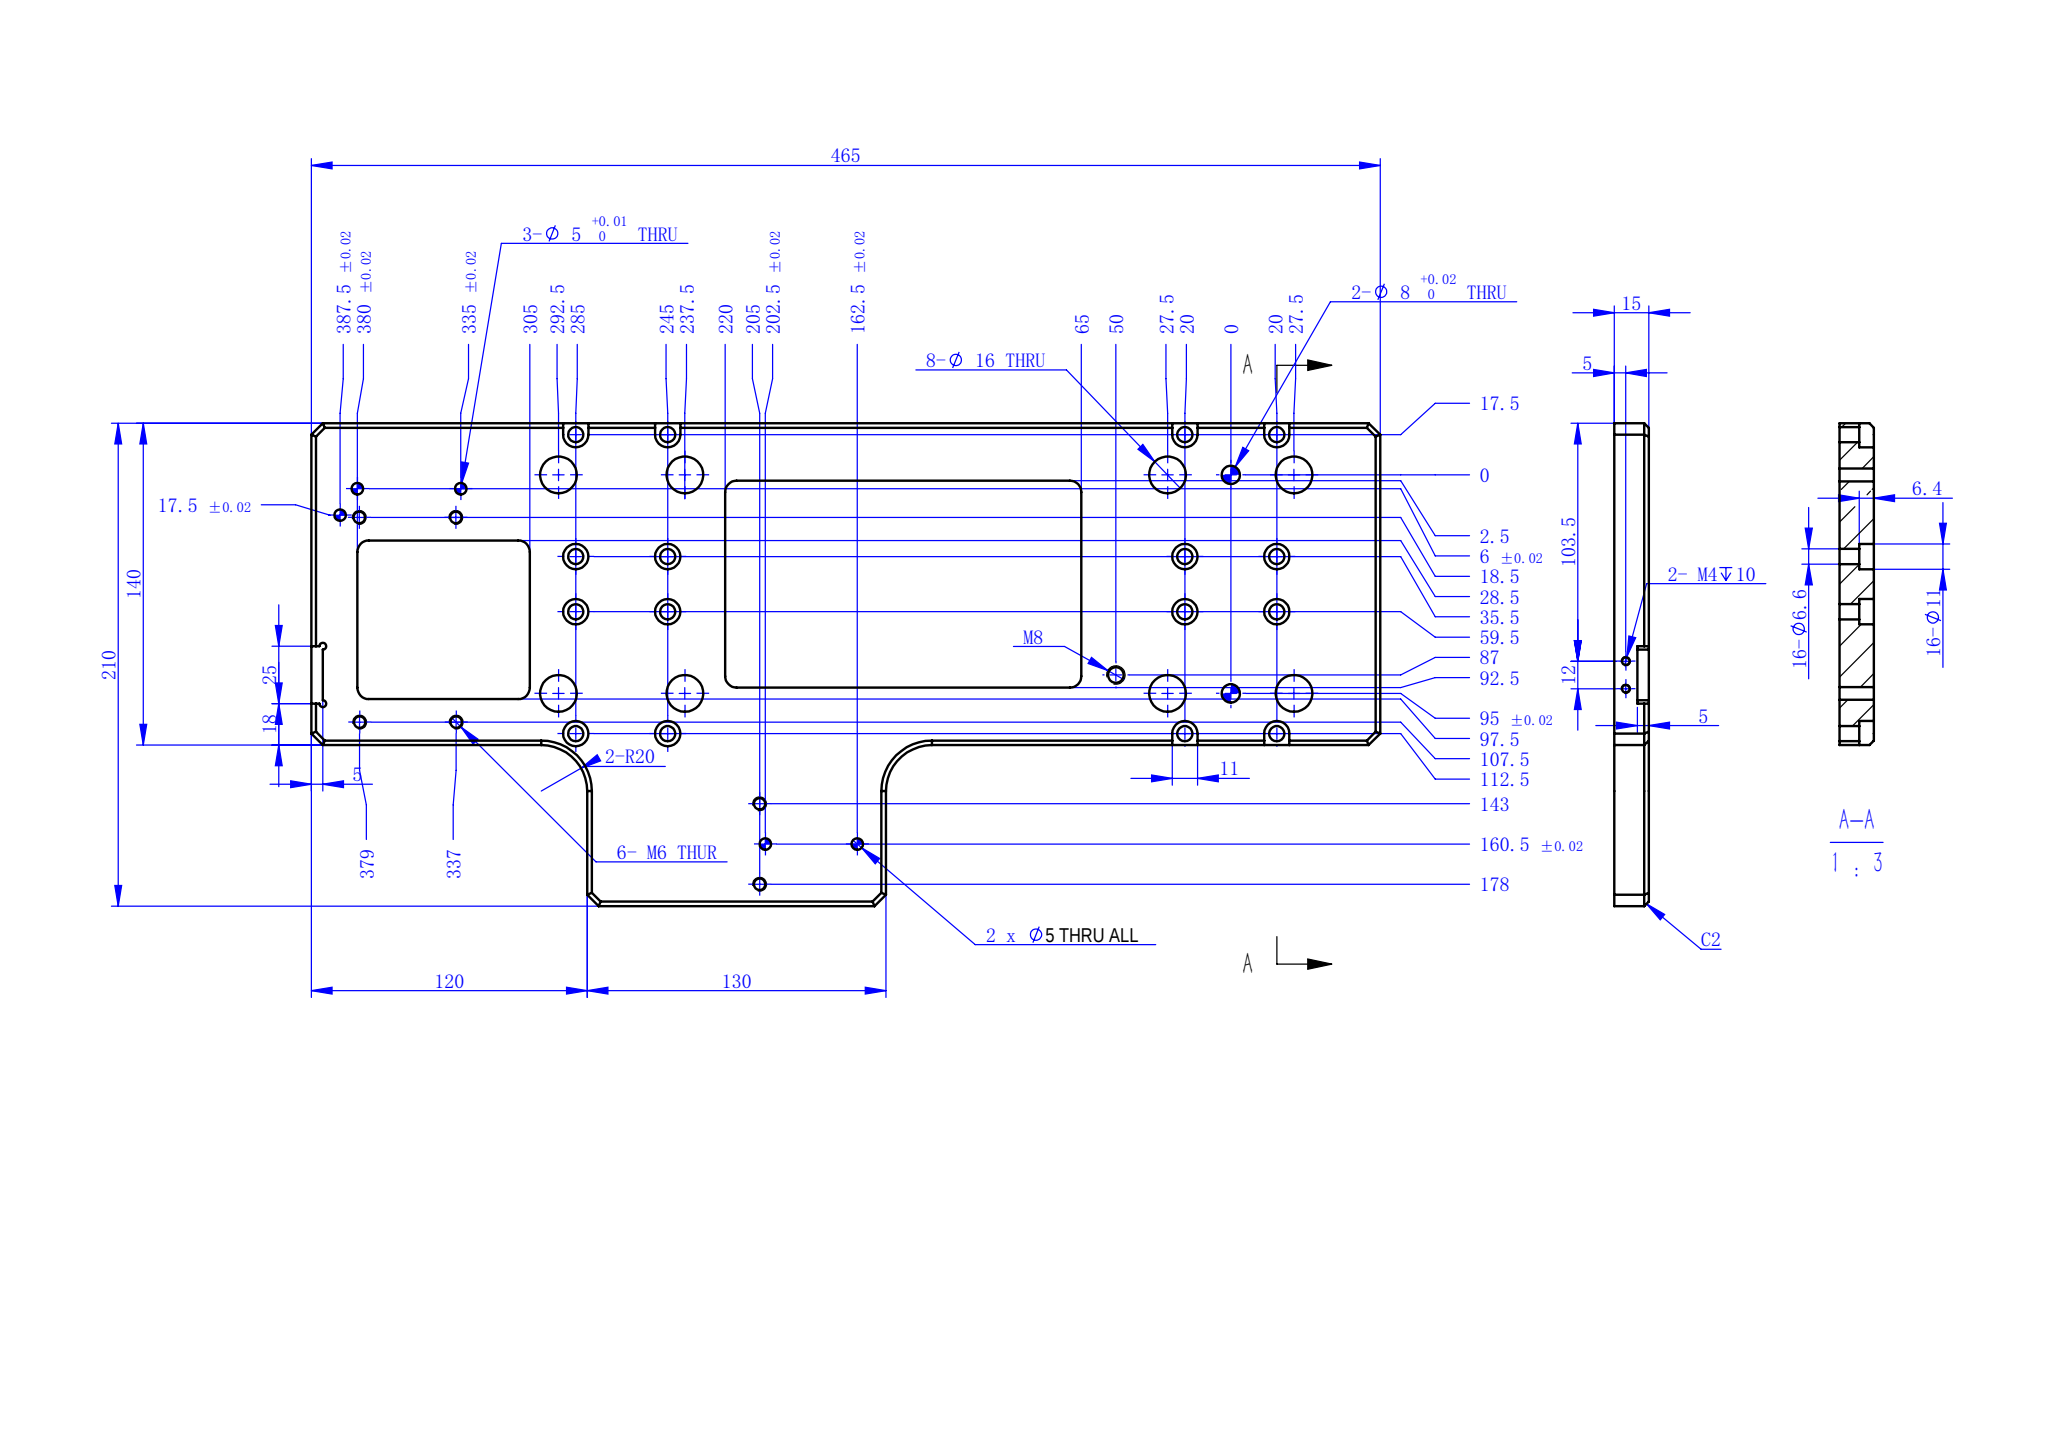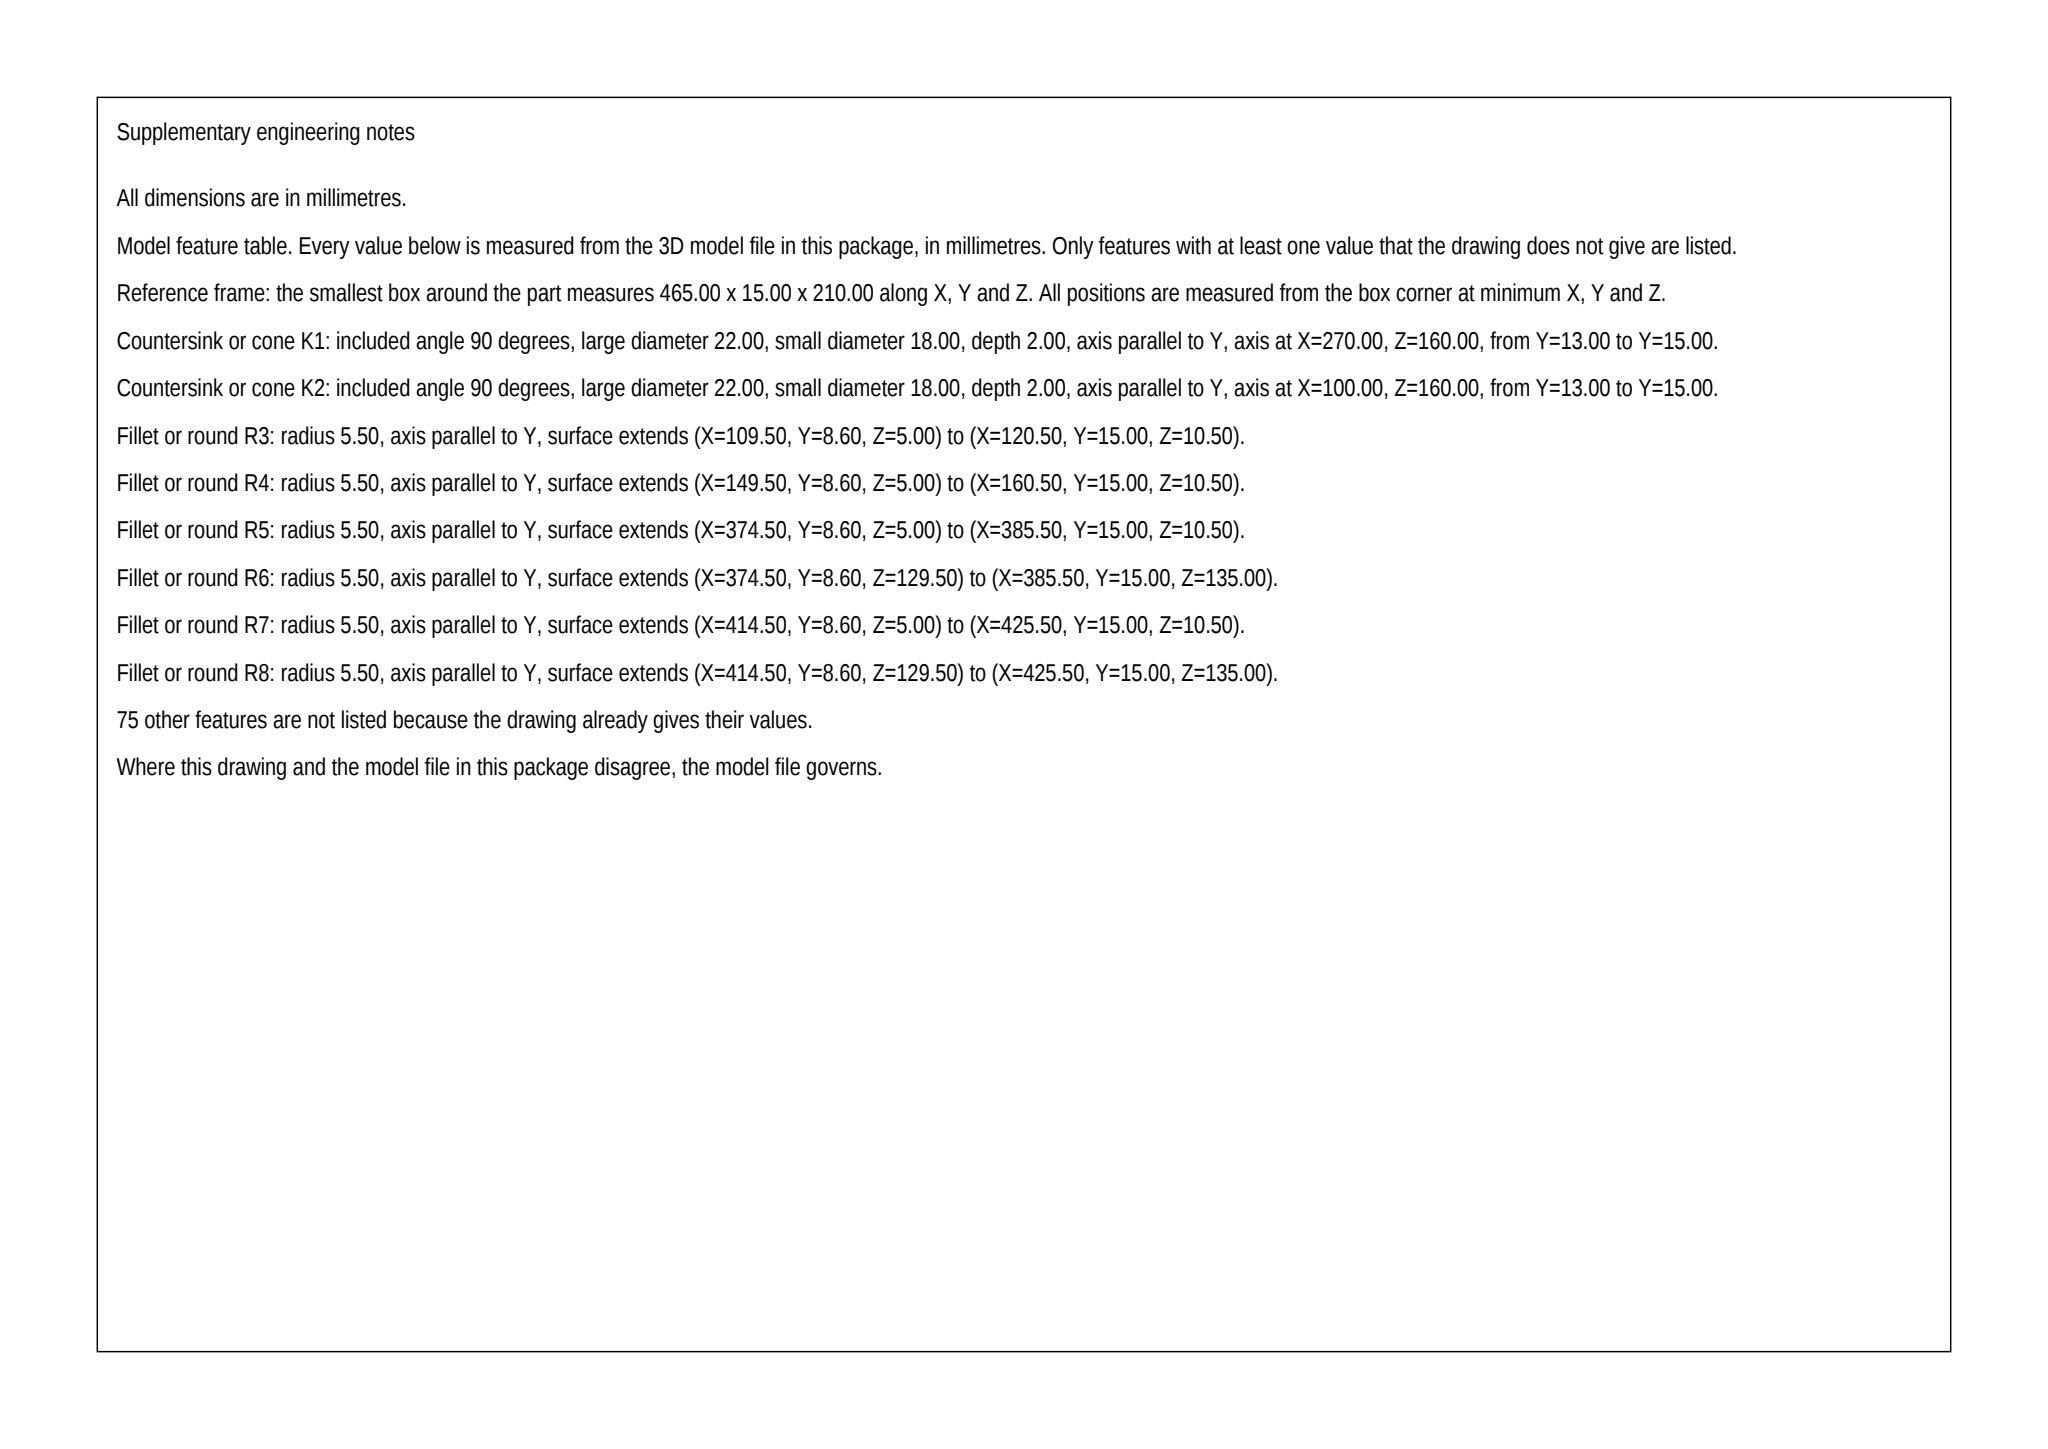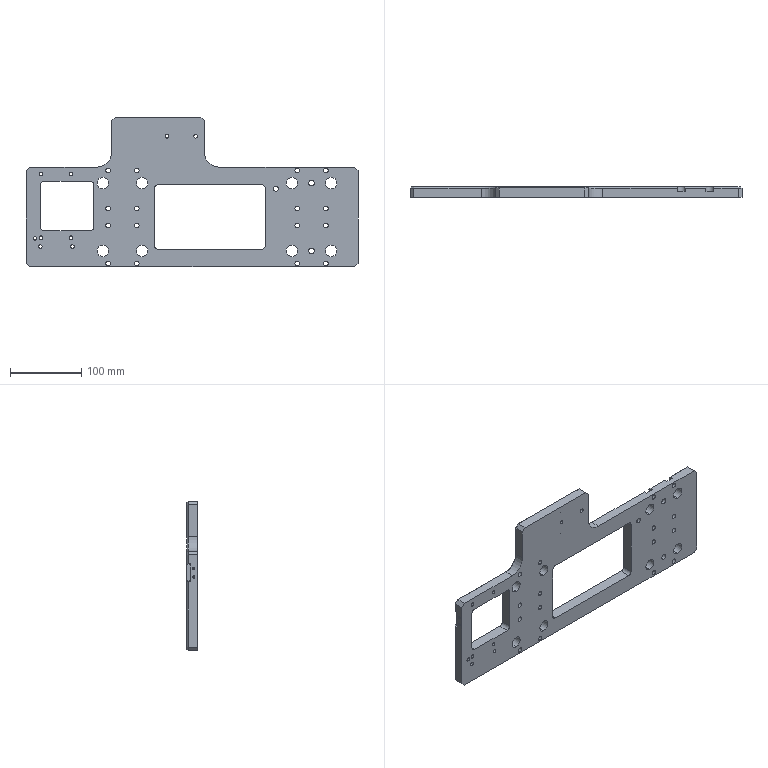Part | SolidWorks | mm | 1 solid | 210 faces | box 465 x 15 x 210 mm | volume 780812 mm3 | cylinder 123 | plane 77 | cone 10 | commonest cylinder face diameters 6.6 x32 11 x30 5 x22 16 x16 10 x8 3.3 x4 8 x4 3 x3
build123d program:
from build123d import *

# Parameters (mm, degrees)
SKETCH1_W                                       = 465
SKETCH1_H                                       = 140
BOSS_EXTRUDE1_DEPTH                             = 15
SKETCH2_W                                       = 130
SKETCH2_H                                       = 15
BOSS_EXTRUDE2_DEPTH                             = 70
FILLET1_R                                       = 20
CHAMFER1_SIZE                                   = 5
CHAMFER2_SIZE                                   = 2
M6_HEX_SOCKET_HEAD_CAP_SCREW_CBORE2_D           = 6.6
M6_HEX_SOCKET_HEAD_CAP_SCREW_CBORE2_CBORE_D     = 11
M6_HEX_SOCKET_HEAD_CAP_SCREW_CBORE2_CBORE_DEPTH = 6.4
SKETCH9_W                                       = 25
SKETCH9_H                                       = 5
CUT_EXTRUDE2_DEPTH                              = 5
SKETCH10_R                                      = 1.5
CUT_EXTRUDE3_DEPTH                              = 5
M8_TAPPED_HOLE1_D                               = 6.8
M6_TAPPED_HOLE3_D                               = 5
SIZE_MM_DOWEL_PIN_HOLE1_D                       = 5
CUT_EXTRUDE4_REACH                              = 273.811
SIZE_MM_DOWEL_PIN_HOLE2_D                       = 8
M6_TAPPED_HOLE4_D                               = 5
M6_TAPPED_HOLE4_DEPTH                           = 13
M6_TAPPED_HOLE4_TIP                             = 1.502
SIZE_MM_DOWEL_PIN_HOLE3_D                       = 5
SKETCH32_W                                      = 155
SKETCH32_H                                      = 90
SKETCH32_W_2                                    = 75
SKETCH32_H_2                                    = 69
CUT_EXTRUDE5_DEPTH                              = 272.811
FILLET2_R                                       = 5
M4_TAPPED_HOLE1_D                               = 3.3
M4_TAPPED_HOLE1_DEPTH                           = 11.5
M4_TAPPED_HOLE1_TIP                             = 0.9914
F_8_0_8_DIAMETER_HOLE1_D                        = 16


with BuildPart() as part:
    # Sketch1 → Boss-Extrude1 (new body)
    with BuildSketch(Plane(origin=(0, 0, 0), x_dir=(1, 0, 0), z_dir=(0, 1, 0))):
        Rectangle(SKETCH1_W, SKETCH1_H)
    extrude(amount=BOSS_EXTRUDE1_DEPTH)

    # Sketch2 → Boss-Extrude2 (add)
    with BuildSketch(Plane.XY.offset(70)):
        with Locations((-47.5, 7.5)):
            Rectangle(SKETCH2_W, SKETCH2_H)
    extrude(amount=BOSS_EXTRUDE2_DEPTH)

    # Fillet1
    fillet1_edges = [part.edges().sort_by_distance(p)[0] for p in [
        (17.5, 7.5, 70),
        (-112.5, 7.5, 70),
    ]]
    fillet(fillet1_edges, radius=FILLET1_R)

    # Chamfer1
    chamfer1_edges = [part.edges().sort_by_distance(p)[0] for p in [
        (-232.5, 7.5, -70),
        (-232.5, 7.5, 70),
        (232.5, 7.5, -70),
        (232.5, 7.5, 70),
        (-112.5, 7.5, 140),
        (17.5, 7.5, 140),
    ]]
    chamfer(chamfer1_edges, length=CHAMFER1_SIZE)

    # Chamfer2
    chamfer2_edges = [part.edges().sort_by_distance(p)[0] for p in [
        (132.5, 15, 70),
        (23.358, 15, 75.858),
        (-118.358, 15, 75.858),
        (-232.5, 15, 0),
        (0, 15, -70),
        (232.5, 15, 0),
        (-180, 15, 70),
        (-112.5, 15, 112.5),
        (-47.5, 15, 140),
        (17.5, 15, 112.5),
        (15, 15, 137.5),
        (-110, 15, 137.5),
        (230, 15, 67.5),
        (230, 15, -67.5),
        (-230, 15, 67.5),
        (-230, 15, -67.5),
    ]]
    chamfer(chamfer2_edges, length=CHAMFER2_SIZE)

    # M6 Hex Socket Head Cap Screw CBORE2 (through all)
    with Locations(Plane(origin=(0, 15, 0), x_dir=(1, 0, 0), z_dir=(0, 1, 0))):
        with Locations((187.5, 65), (147.5, 65), (147.5, 12), (187.5, 12), (187.5, -12), (147.5, -12), (147.5, -65), (187.5, -65), (-117.5, 65), (-77.5, 65), (-117.5, -65), (-77.5, -65), (-77.5, -12), (-117.5, -12), (-117.5, 12), (-77.5, 12)):
            CounterBoreHole(M6_HEX_SOCKET_HEAD_CAP_SCREW_CBORE2_D / 2, M6_HEX_SOCKET_HEAD_CAP_SCREW_CBORE2_CBORE_D / 2, M6_HEX_SOCKET_HEAD_CAP_SCREW_CBORE2_CBORE_DEPTH)

    # Sketch9 → Cut-Extrude2 (cut)
    with BuildSketch(Plane.ZY.offset(232.5)):
        with Locations((39.5, 12.5)):
            Rectangle(SKETCH9_W, SKETCH9_H)
    extrude(amount=-CUT_EXTRUDE2_DEPTH, mode=Mode.SUBTRACT)

    # Sketch10 → Cut-Extrude3 (cut)
    with BuildSketch(Plane(origin=(0, 15, 0), x_dir=(1, 0, 0), z_dir=(0, 1, 0))):
        with Locations((-227.5, -27)):
            Circle(SKETCH10_R)
        with Locations((-227.5, -52)):
            Circle(SKETCH10_R)
    extrude(amount=-CUT_EXTRUDE3_DEPTH, mode=Mode.SUBTRACT)

    # M8 Tapped Hole1 (through all)
    with Locations(Plane(origin=(0, 0, 0), x_dir=(-1, 0, 0), z_dir=(0, -1, 0))):
        with Locations((-117.5, -39.5)):
            Hole(M8_TAPPED_HOLE1_D / 2)

    # M6 Tapped Hole3 (through all)
    with Locations(Plane(origin=(0, 15, 0), x_dir=(1, 0, 0), z_dir=(0, 1, 0))):
        with Locations((-169.5, -60), (-211.5, -60), (-211.666, 29), (-169.666, 29)):
            Hole(M6_TAPPED_HOLE3_D / 2)

    # Size mm Dowel Pin Hole1 (through all)
    with Locations(Plane(origin=(0, 15, 0), x_dir=(1, 0, 0), z_dir=(0, 1, 0))):
        with Locations((-212.5, 41.5), (-167.5, 41.5), (-220, 30)):
            Hole(SIZE_MM_DOWEL_PIN_HOLE1_D / 2)

    # Cut-Extrude4: up to this face of the body (flat: up to its plane)
    cut_extrude4_end = Plane(part.part.faces().sort_by_distance((147.5, 8.6, -69.848))[0])
    # Sketch24 → Cut-Extrude4 (cut, up to the picked face)
    with BuildSketch(Plane(origin=(0, 15, 0), x_dir=(1, 0, 0), z_dir=(0, 1, 0)), mode=Mode.PRIVATE) as cut_extrude4_sk1:
        with BuildLine():
            Line((193, -65), (193, -78.407))
            ThreePointArc((193, -78.407), (187.5, -83.907), (182, -78.407))
            Line((182, -78.407), (182, -65))
            ThreePointArc((182, -65), (187.5, -59.5), (193, -65))
        make_face()
    cut_extrude4_tool1 = split(extrude(cut_extrude4_sk1.sketch, amount=-CUT_EXTRUDE4_REACH, mode=Mode.PRIVATE), bisect_by=cut_extrude4_end, keep=Keep.BOTH, mode=Mode.PRIVATE)
    # Sketch24 → Cut-Extrude4 (cut, up to the picked face)
    with BuildSketch(Plane(origin=(0, 15, 0), x_dir=(1, 0, 0), z_dir=(0, 1, 0)), mode=Mode.PRIVATE) as cut_extrude4_sk2:
        with BuildLine():
            Line((153, -65), (153, -78.407))
            ThreePointArc((153, -78.407), (147.5, -83.907), (142, -78.407))
            Line((142, -78.407), (142, -65))
            ThreePointArc((142, -65), (147.5, -59.5), (153, -65))
        make_face()
    cut_extrude4_tool2 = split(extrude(cut_extrude4_sk2.sketch, amount=-CUT_EXTRUDE4_REACH, mode=Mode.PRIVATE), bisect_by=cut_extrude4_end, keep=Keep.BOTH, mode=Mode.PRIVATE)
    # Sketch24 → Cut-Extrude4 (cut, up to the picked face)
    with BuildSketch(Plane(origin=(0, 15, 0), x_dir=(1, 0, 0), z_dir=(0, 1, 0)), mode=Mode.PRIVATE) as cut_extrude4_sk3:
        with BuildLine():
            Line((182, 65), (182, 76.928))
            ThreePointArc((182, 76.928), (187.5, 82.428), (193, 76.928))
            Line((193, 76.928), (193, 65))
            ThreePointArc((193, 65), (187.5, 59.5), (182, 65))
        make_face()
    cut_extrude4_tool3 = split(extrude(cut_extrude4_sk3.sketch, amount=-CUT_EXTRUDE4_REACH, mode=Mode.PRIVATE), bisect_by=cut_extrude4_end, keep=Keep.BOTH, mode=Mode.PRIVATE)
    # Sketch24 → Cut-Extrude4 (cut, up to the picked face)
    with BuildSketch(Plane(origin=(0, 15, 0), x_dir=(1, 0, 0), z_dir=(0, 1, 0)), mode=Mode.PRIVATE) as cut_extrude4_sk4:
        with BuildLine():
            Line((142, 65), (142, 76.928))
            ThreePointArc((142, 76.928), (147.5, 82.428), (153, 76.928))
            Line((153, 76.928), (153, 65))
            ThreePointArc((153, 65), (147.5, 59.5), (142, 65))
        make_face()
    cut_extrude4_tool4 = split(extrude(cut_extrude4_sk4.sketch, amount=-CUT_EXTRUDE4_REACH, mode=Mode.PRIVATE), bisect_by=cut_extrude4_end, keep=Keep.BOTH, mode=Mode.PRIVATE)
    # Sketch24 → Cut-Extrude4 (cut, up to the picked face)
    with BuildSketch(Plane(origin=(0, 15, 0), x_dir=(1, 0, 0), z_dir=(0, 1, 0)), mode=Mode.PRIVATE) as cut_extrude4_sk5:
        with BuildLine():
            Line((-83, 65), (-83, 75.208))
            ThreePointArc((-83, 75.208), (-77.5, 80.708), (-72, 75.208))
            Line((-72, 75.208), (-72, 65))
            ThreePointArc((-72, 65), (-77.5, 59.5), (-83, 65))
        make_face()
    cut_extrude4_tool5 = split(extrude(cut_extrude4_sk5.sketch, amount=-CUT_EXTRUDE4_REACH, mode=Mode.PRIVATE), bisect_by=cut_extrude4_end, keep=Keep.BOTH, mode=Mode.PRIVATE)
    # Sketch24 → Cut-Extrude4 (cut, up to the picked face)
    with BuildSketch(Plane(origin=(0, 15, 0), x_dir=(1, 0, 0), z_dir=(0, 1, 0)), mode=Mode.PRIVATE) as cut_extrude4_sk6:
        with BuildLine():
            Line((-123, 65), (-123, 75.208))
            ThreePointArc((-123, 75.208), (-117.5, 80.708), (-112, 75.208))
            Line((-112, 75.208), (-112, 65))
            ThreePointArc((-112, 65), (-117.5, 59.5), (-123, 65))
        make_face()
    cut_extrude4_tool6 = split(extrude(cut_extrude4_sk6.sketch, amount=-CUT_EXTRUDE4_REACH, mode=Mode.PRIVATE), bisect_by=cut_extrude4_end, keep=Keep.BOTH, mode=Mode.PRIVATE)
    add(cut_extrude4_tool1.solids().sort_by(Axis((187.5, 15, 71.703), (0, -1, 0)))[0], mode=Mode.SUBTRACT)
    add(cut_extrude4_tool2.solids().sort_by(Axis((147.5, 15, 71.703), (0, -1, 0)))[0], mode=Mode.SUBTRACT)
    add(cut_extrude4_tool3.solids().sort_by(Axis((187.5, 15, -70.964), (0, -1, 0)))[0], mode=Mode.SUBTRACT)
    add(cut_extrude4_tool4.solids().sort_by(Axis((147.5, 15, -70.964), (0, -1, 0)))[0], mode=Mode.SUBTRACT)
    add(cut_extrude4_tool5.solids().sort_by(Axis((-77.5, 15, -70.104), (0, -1, 0)))[0], mode=Mode.SUBTRACT)
    add(cut_extrude4_tool6.solids().sort_by(Axis((-117.5, 15, -70.104), (0, -1, 0)))[0], mode=Mode.SUBTRACT)

    # Size mm Dowel Pin Hole2 (through all)
    with Locations(Plane(origin=(0, 15, 0), x_dir=(1, 0, 0), z_dir=(0, 1, 0))):
        with Locations((167.5, 47.5), (167.5, -47.5)):
            Hole(SIZE_MM_DOWEL_PIN_HOLE2_D / 2)

    # M6 Tapped Hole4
    with Locations(Plane(origin=(0, 15, 0), x_dir=(1, 0, 0), z_dir=(0, 1, 0))):
        with Locations((-37.5, -95.5), (-37.5, -130.5)):
            Hole(M6_TAPPED_HOLE4_D / 2, depth=M6_TAPPED_HOLE4_DEPTH)
            with Locations((0, 0, -(M6_TAPPED_HOLE4_DEPTH + M6_TAPPED_HOLE4_TIP / 2))):  # 118° drill point
                Cone(0, M6_TAPPED_HOLE4_D / 2, M6_TAPPED_HOLE4_TIP, mode=Mode.SUBTRACT)

    # Size mm Dowel Pin Hole3 (through all)
    with Locations(Plane(origin=(0, 15, 0), x_dir=(1, 0, 0), z_dir=(0, 1, 0))):
        with Locations((-35, -113), (5, -113)):
            Hole(SIZE_MM_DOWEL_PIN_HOLE3_D / 2)

    # Sketch32 → Cut-Extrude5 (cut, through all)
    with BuildSketch(Plane(origin=(0, 15, 0), x_dir=(1, 0, 0), z_dir=(0, 1, 0))):
        with Locations((25, 0)):
            Rectangle(SKETCH32_W, SKETCH32_H)
        with Locations((-175, -15.5)):
            Rectangle(SKETCH32_W_2, SKETCH32_H_2)
    extrude(amount=-CUT_EXTRUDE5_DEPTH, mode=Mode.SUBTRACT)

    # Fillet2
    fillet2_edges = [part.edges().sort_by_distance(p)[0] for p in [
        (102.5, 7.5, -45),
        (102.5, 7.5, 45),
        (-52.5, 7.5, 45),
        (-52.5, 7.5, -45),
        (-212.5, 7.5, 50),
        (-212.5, 7.5, -19),
        (-137.5, 7.5, -19),
        (-137.5, 7.5, 50),
    ]]
    fillet(fillet2_edges, radius=FILLET2_R)

    # M4 Tapped Hole1
    with Locations(Plane.ZY.offset(232.5)):
        with Locations((33.5, 5), (45.5, 5)):
            Hole(M4_TAPPED_HOLE1_D / 2, depth=M4_TAPPED_HOLE1_DEPTH)
            with Locations((0, 0, -(M4_TAPPED_HOLE1_DEPTH + M4_TAPPED_HOLE1_TIP / 2))):  # 118° drill point
                Cone(0, M4_TAPPED_HOLE1_D / 2, M4_TAPPED_HOLE1_TIP, mode=Mode.SUBTRACT)

    # 8.0 _8_ Diameter Hole1 (through all)
    with Locations(Plane(origin=(0, 15, 0), x_dir=(1, 0, 0), z_dir=(0, 1, 0))):
        with Locations((195, -47.5), (140, -47.5), (195, 47.5), (140, 47.5), (-70, -47.5), (-125, -47.5), (-70, 47.5), (-125, 47.5)):
            Hole(F_8_0_8_DIAMETER_HOLE1_D / 2)


solid = part.part